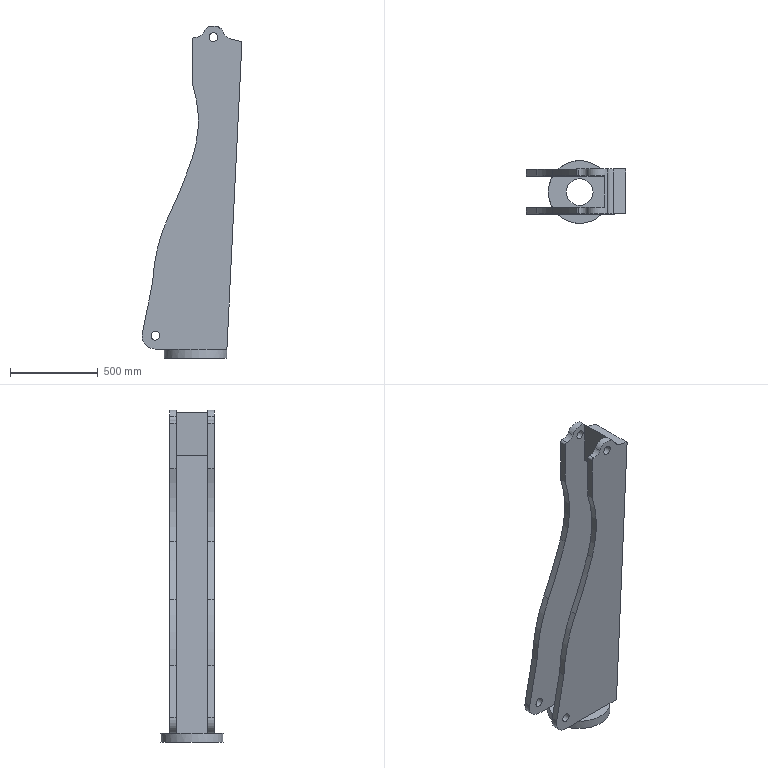Component | NX | SUPPORT_ARM | 1 solid | 46 faces | volume 63328619 mm3 | plane 24 | cylinder 22 | commonest cylinder face diameters 50.8 x4 100 x3 150 x2 2031.109 x2 5409.506 x2 1313.552 x2 25.4 x2 127 x1